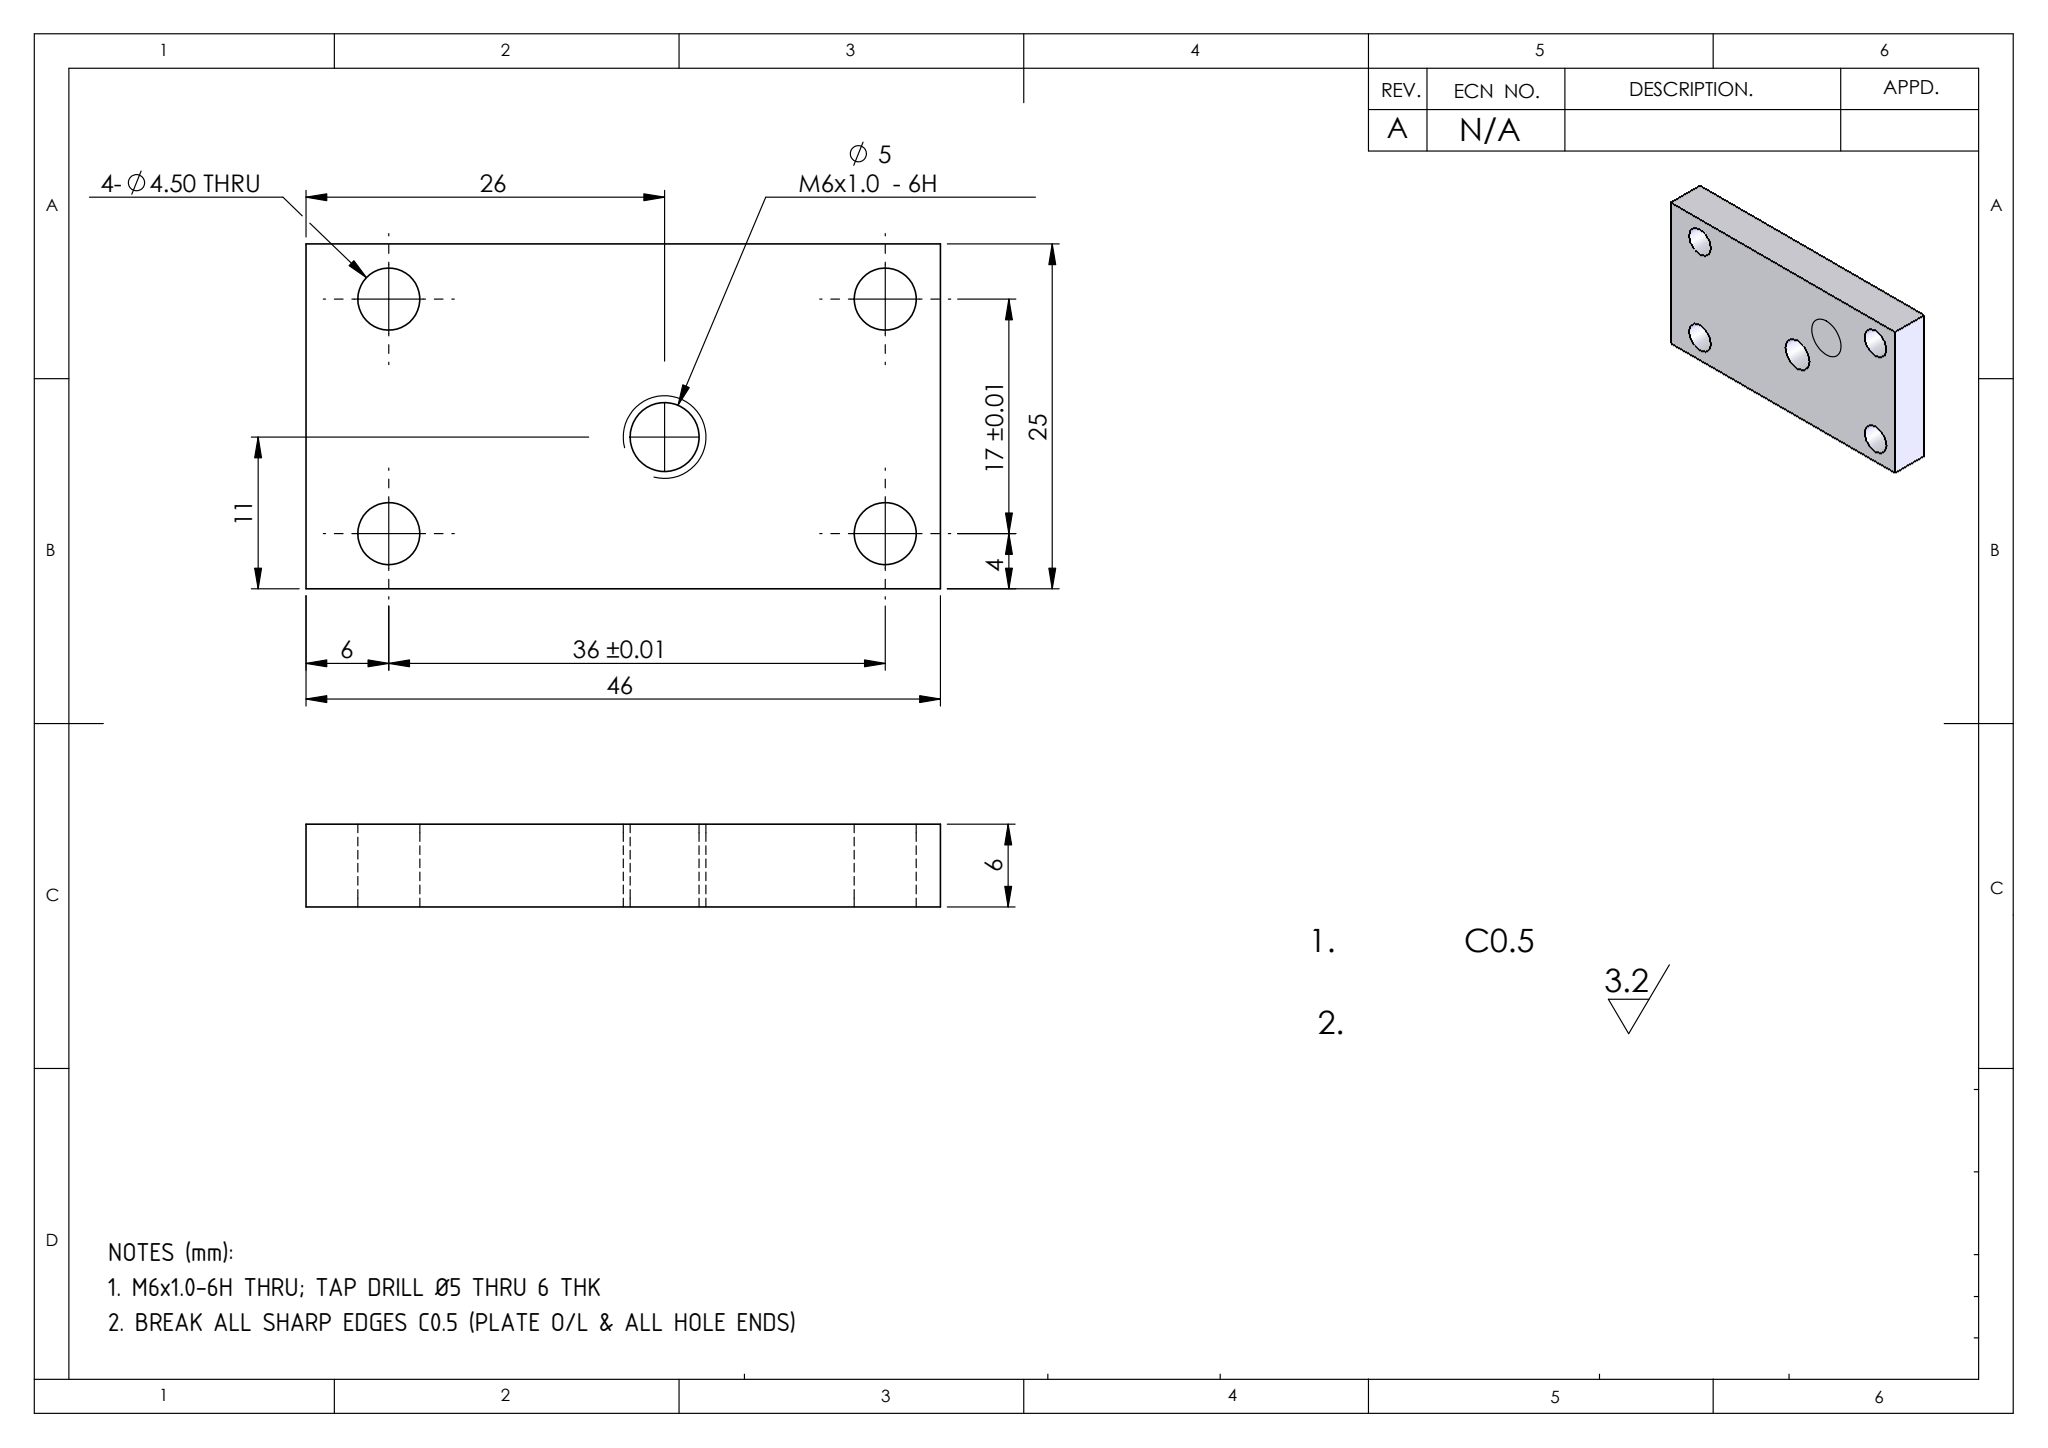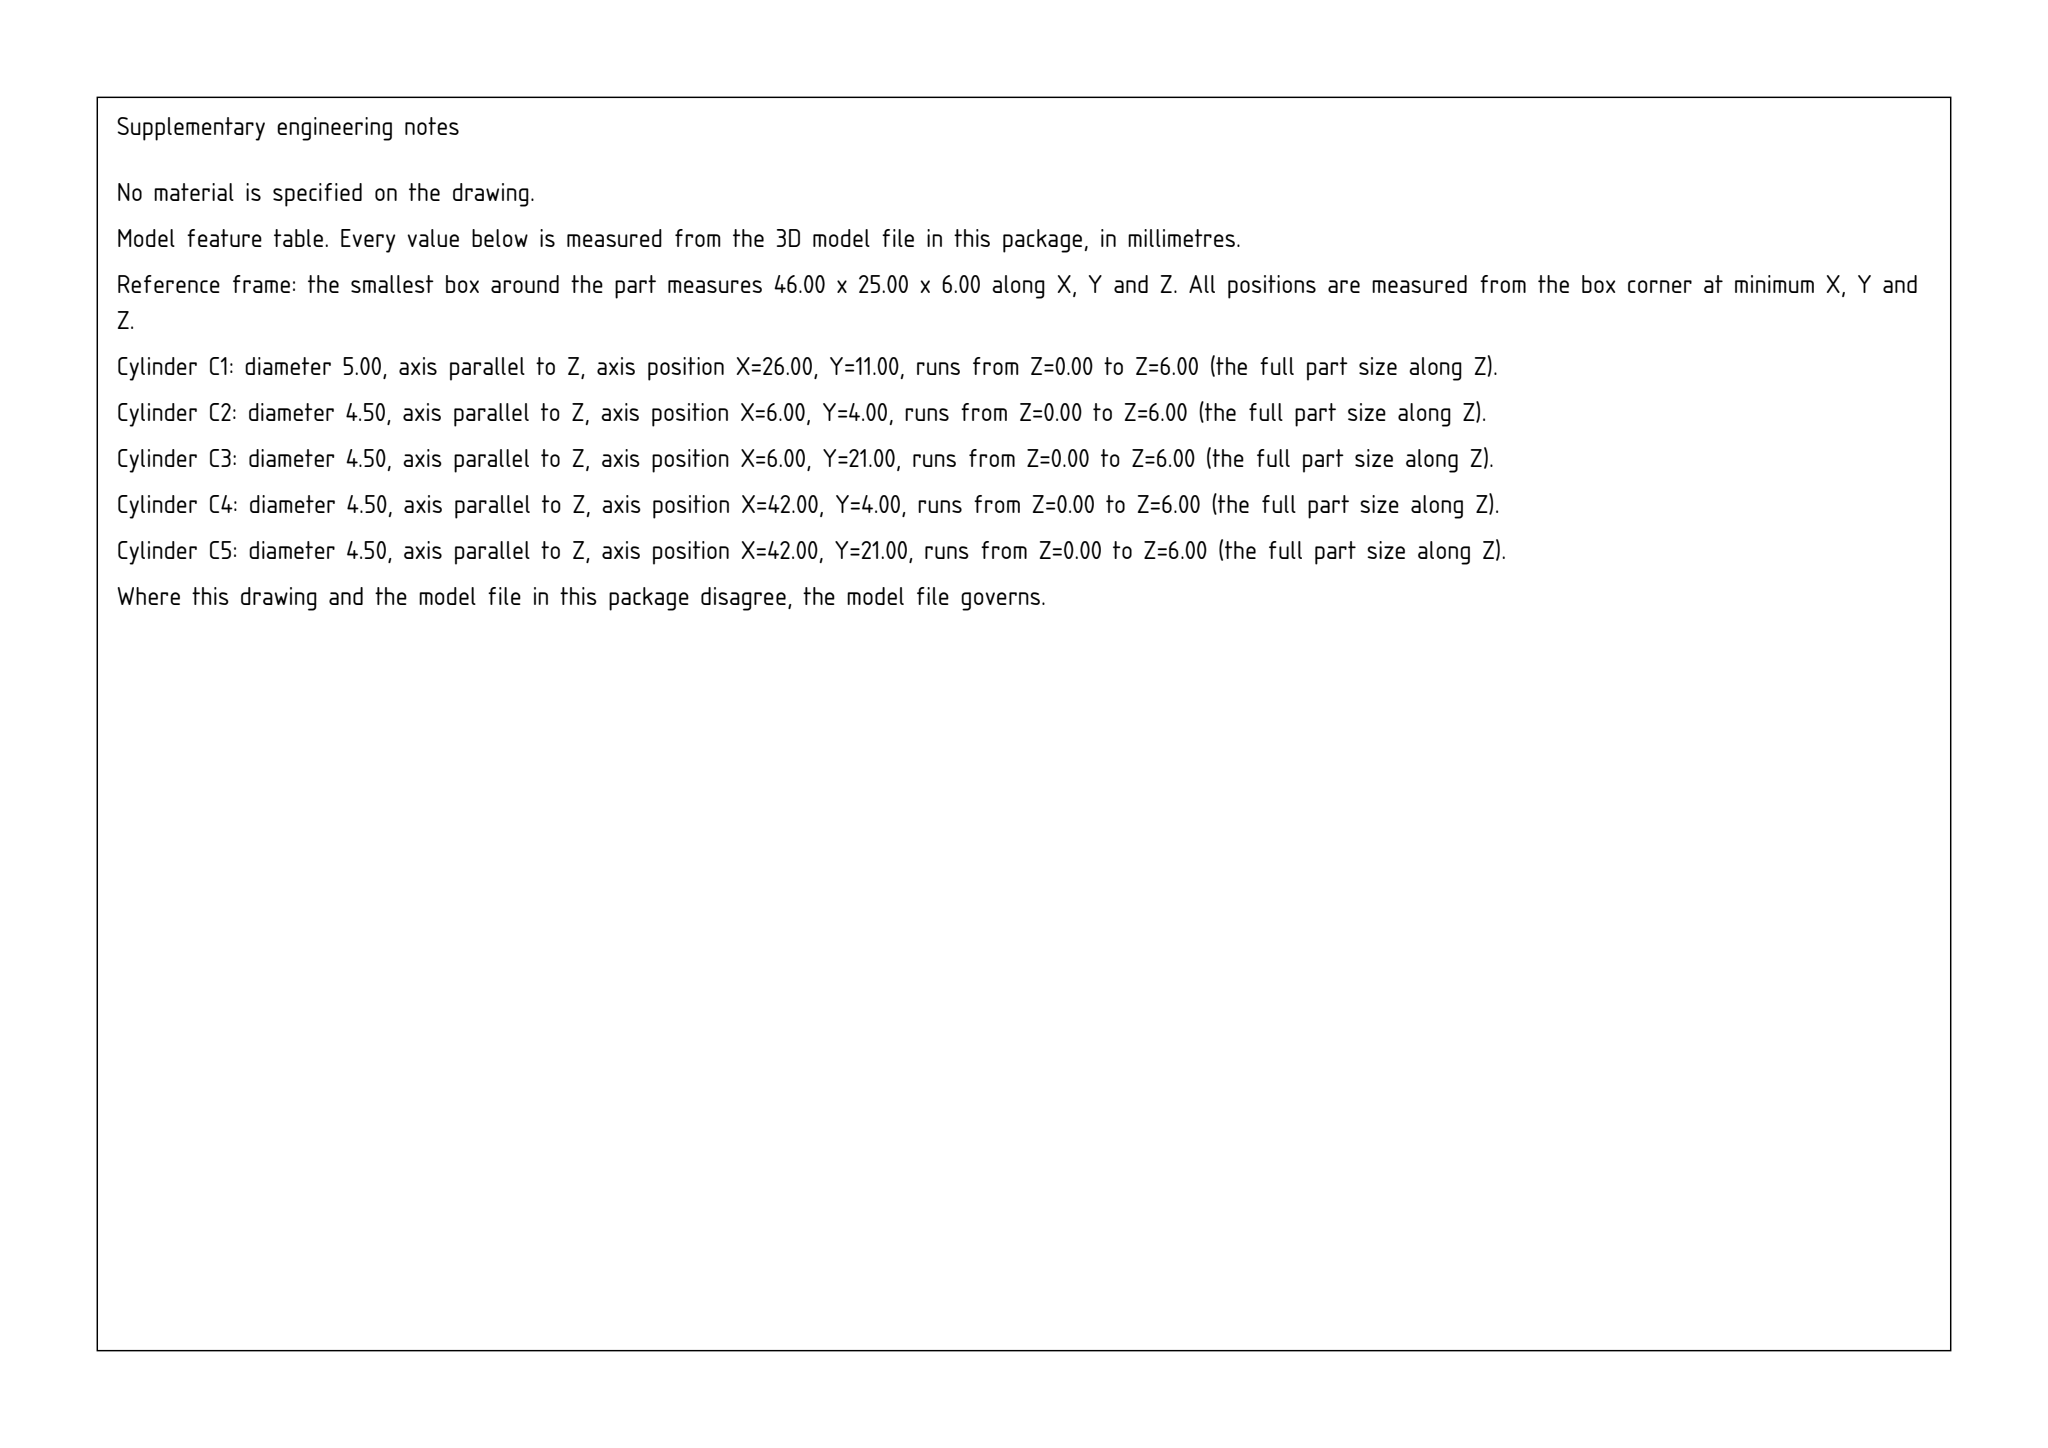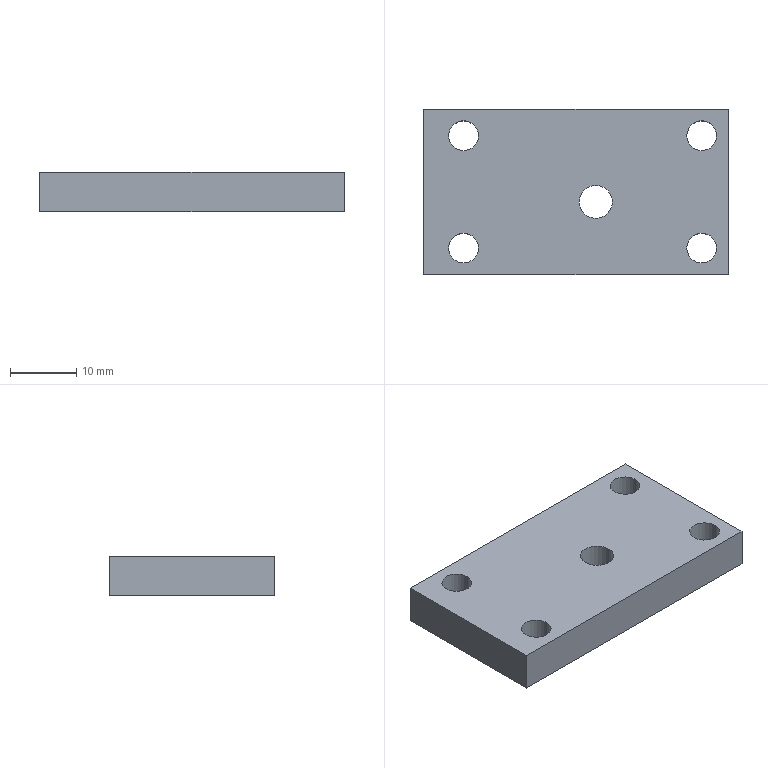Part | SolidWorks | mm | 1 solid | 16 faces | box 46 x 25 x 6 mm | volume 6400 mm3 | cylinder 10 | plane 6 | commonest cylinder face diameters 4.5 x8 5 x2
Drawing notes:
M6x1.0-6H THRU; TAP DRILL Ø5 THRU 6 THK | from the solid: Ø5 cylinder, axis z, at (26,11), length 6 = full plate thk (bbox z=6)
BREAK ALL SHARP EDGES C0.5 (PLATE O/L & ALL HOLE ENDS) | from the solid: No chamfer/fillet features in STEP; all 6 planar faces & 5 thru-hole ends meet sharp
build123d program:
from build123d import *

# Parameters (mm, degrees)
SKETCH1_W          = 46
SKETCH1_H          = 25
EXTRUDE1_DEPTH     = 6
SKETCH2_R          = 2.25
CUT_EXTRUDE1_DEPTH = 10
M6_TAPPED_HOLE1_D  = 5


with BuildPart() as part:
    # Sketch1 → Extrude1 (new body)
    with BuildSketch(Plane.XY):
        Rectangle(SKETCH1_W, SKETCH1_H)
    extrude(amount=EXTRUDE1_DEPTH)

    # Sketch2 → Cut-Extrude1 (cut)
    with BuildSketch(Plane(origin=(0, 0, 0), x_dir=(-1, 0, 0), z_dir=(0, 0, -1))):
        with Locations((-19, 8.5)):
            Circle(SKETCH2_R)
        with Locations((17, 8.5)):
            Circle(SKETCH2_R)
        with Locations((17, -8.5)):
            Circle(SKETCH2_R)
        with Locations((-19, -8.5)):
            Circle(SKETCH2_R)
    extrude(amount=-CUT_EXTRUDE1_DEPTH, mode=Mode.SUBTRACT)

    # M6 Tapped Hole1 (through all)
    with Locations(Plane(origin=(3, -1.5, 0), x_dir=(-1, 0, 0), z_dir=(0, 0, -1))):
        with Locations((0, 0)):
            Hole(M6_TAPPED_HOLE1_D / 2)


solid = part.part
STEP:
#1=CARTESIAN_POINT('',(5.5,-1.5,6.));
#2=VERTEX_POINT('',#1);
#3=CARTESIAN_POINT('',(0.5,-1.5,6.));
#4=VERTEX_POINT('',#3);
#5=CARTESIAN_POINT('',(3.,-1.5,6.));
#6=DIRECTION('',(0.,0.,-1.));
#7=DIRECTION('',(-1.,0.,0.));
#8=AXIS2_PLACEMENT_3D('',#5,#6,#7);
#9=CIRCLE('',#8,2.5);
#10=EDGE_CURVE('',#2,#4,#9,.T.);
#11=ORIENTED_EDGE('',*,*,#10,.F.);
#12=CARTESIAN_POINT('',(5.5,-1.5,0.));
#13=VERTEX_POINT('',#12);
#14=CARTESIAN_POINT('',(5.5,-1.5,-0.));
#15=DIRECTION('',(0.,0.,-1.));
#16=VECTOR('',#15,1000.);
#17=LINE('',#14,#16);
#18=EDGE_CURVE('',#2,#13,#17,.T.);
#19=ORIENTED_EDGE('',*,*,#18,.T.);
#20=CARTESIAN_POINT('',(0.5,-1.5,0.));
#21=VERTEX_POINT('',#20);
#22=CARTESIAN_POINT('',(3.,-1.5,0.));
#23=DIRECTION('',(0.,0.,-1.));
#24=DIRECTION('',(-1.,0.,0.));
#25=AXIS2_PLACEMENT_3D('',#22,#23,#24);
#26=CIRCLE('',#25,2.5);
#27=EDGE_CURVE('',#13,#21,#26,.T.);
#28=ORIENTED_EDGE('',*,*,#27,.T.);
#29=CARTESIAN_POINT('',(0.5,-1.5,0.));
#30=DIRECTION('',(0.,0.,-1.));
#31=VECTOR('',#30,1000.);
#32=LINE('',#29,#31);
#33=EDGE_CURVE('',#4,#21,#32,.T.);
#34=ORIENTED_EDGE('',*,*,#33,.F.);
#35=EDGE_LOOP('',(#11,#19,#28,#34));
#36=FACE_OUTER_BOUND('',#35,.T.);
#37=CARTESIAN_POINT('',(3.,-1.5,0.));
#38=DIRECTION('',(0.,0.,-1.));
#39=DIRECTION('',(-1.,0.,0.));
#40=AXIS2_PLACEMENT_3D('',#37,#38,#39);
#41=CYLINDRICAL_SURFACE('',#40,2.5);
#42=ADVANCED_FACE('',(#36),#41,.F.);
#43=CARTESIAN_POINT('',(21.25,-8.5,6.));
#44=VERTEX_POINT('',#43);
#45=CARTESIAN_POINT('',(16.75,-8.5,6.));
#46=VERTEX_POINT('',#45);
#47=CARTESIAN_POINT('',(19.,-8.5,6.));
#48=DIRECTION('',(0.,0.,-1.));
#49=DIRECTION('',(-1.,0.,0.));
#50=AXIS2_PLACEMENT_3D('',#47,#48,#49);
#51=CIRCLE('',#50,2.25);
#52=EDGE_CURVE('',#44,#46,#51,.T.);
#53=ORIENTED_EDGE('',*,*,#52,.F.);
#54=CARTESIAN_POINT('',(21.25,-8.5,0.));
#55=VERTEX_POINT('',#54);
#56=CARTESIAN_POINT('',(21.25,-8.5,10.));
#57=DIRECTION('',(0.,0.,-1.));
#58=VECTOR('',#57,1000.);
#59=LINE('',#56,#58);
#60=EDGE_CURVE('',#44,#55,#59,.T.);
#61=ORIENTED_EDGE('',*,*,#60,.T.);
#62=CARTESIAN_POINT('',(16.75,-8.5,-0.));
#63=VERTEX_POINT('',#62);
#64=CARTESIAN_POINT('',(19.,-8.5,0.));
#65=DIRECTION('',(0.,0.,-1.));
#66=DIRECTION('',(1.,0.,-0.));
#67=AXIS2_PLACEMENT_3D('',#64,#65,#66);
#68=CIRCLE('',#67,2.25);
#69=EDGE_CURVE('',#55,#63,#68,.T.);
#70=ORIENTED_EDGE('',*,*,#69,.T.);
#71=CARTESIAN_POINT('',(16.75,-8.5,10.));
#72=DIRECTION('',(0.,0.,-1.));
#73=VECTOR('',#72,1000.);
#74=LINE('',#71,#73);
#75=EDGE_CURVE('',#46,#63,#74,.T.);
#76=ORIENTED_EDGE('',*,*,#75,.F.);
#77=EDGE_LOOP('',(#53,#61,#70,#76));
#78=FACE_OUTER_BOUND('',#77,.T.);
#79=CARTESIAN_POINT('',(19.,-8.5,10.));
#80=DIRECTION('',(0.,0.,-1.));
#81=DIRECTION('',(-1.,0.,0.));
#82=AXIS2_PLACEMENT_3D('',#79,#80,#81);
#83=CYLINDRICAL_SURFACE('',#82,2.25);
#84=ADVANCED_FACE('',(#78),#83,.F.);
#85=CARTESIAN_POINT('',(-14.75,-8.5,6.));
#86=VERTEX_POINT('',#85);
#87=CARTESIAN_POINT('',(-19.25,-8.5,6.));
#88=VERTEX_POINT('',#87);
#89=CARTESIAN_POINT('',(-17.,-8.5,6.));
#90=DIRECTION('',(0.,0.,-1.));
#91=DIRECTION('',(-1.,0.,0.));
#92=AXIS2_PLACEMENT_3D('',#89,#90,#91);
#93=CIRCLE('',#92,2.25);
#94=EDGE_CURVE('',#86,#88,#93,.T.);
#95=ORIENTED_EDGE('',*,*,#94,.F.);
#96=CARTESIAN_POINT('',(-14.75,-8.5,0.));
#97=VERTEX_POINT('',#96);
#98=CARTESIAN_POINT('',(-14.75,-8.5,10.));
#99=DIRECTION('',(0.,0.,-1.));
#100=VECTOR('',#99,1000.);
#101=LINE('',#98,#100);
#102=EDGE_CURVE('',#86,#97,#101,.T.);
#103=ORIENTED_EDGE('',*,*,#102,.T.);
#104=CARTESIAN_POINT('',(-19.25,-8.5,0.));
#105=VERTEX_POINT('',#104);
#106=CARTESIAN_POINT('',(-17.,-8.5,0.));
#107=DIRECTION('',(0.,0.,-1.));
#108=DIRECTION('',(1.,0.,-0.));
#109=AXIS2_PLACEMENT_3D('',#106,#107,#108);
#110=CIRCLE('',#109,2.25);
#111=EDGE_CURVE('',#97,#105,#110,.T.);
#112=ORIENTED_EDGE('',*,*,#111,.T.);
#113=CARTESIAN_POINT('',(-19.25,-8.5,10.));
#114=DIRECTION('',(0.,0.,-1.));
#115=VECTOR('',#114,1000.);
#116=LINE('',#113,#115);
#117=EDGE_CURVE('',#88,#105,#116,.T.);
#118=ORIENTED_EDGE('',*,*,#117,.F.);
#119=EDGE_LOOP('',(#95,#103,#112,#118));
#120=FACE_OUTER_BOUND('',#119,.T.);
#121=CARTESIAN_POINT('',(-17.,-8.5,10.));
#122=DIRECTION('',(0.,0.,-1.));
#123=DIRECTION('',(-1.,0.,0.));
#124=AXIS2_PLACEMENT_3D('',#121,#122,#123);
#125=CYLINDRICAL_SURFACE('',#124,2.25);
#126=ADVANCED_FACE('',(#120),#125,.F.);
#127=CARTESIAN_POINT('',(-14.75,8.5,6.));
#128=VERTEX_POINT('',#127);
#129=CARTESIAN_POINT('',(-19.25,8.5,6.));
#130=VERTEX_POINT('',#129);
#131=CARTESIAN_POINT('',(-17.,8.5,6.));
#132=DIRECTION('',(0.,0.,-1.));
#133=DIRECTION('',(-1.,0.,0.));
#134=AXIS2_PLACEMENT_3D('',#131,#132,#133);
#135=CIRCLE('',#134,2.25);
#136=EDGE_CURVE('',#128,#130,#135,.T.);
#137=ORIENTED_EDGE('',*,*,#136,.F.);
#138=CARTESIAN_POINT('',(-14.75,8.5,0.));
#139=VERTEX_POINT('',#138);
#140=CARTESIAN_POINT('',(-14.75,8.5,10.));
#141=DIRECTION('',(0.,0.,-1.));
#142=VECTOR('',#141,1000.);
#143=LINE('',#140,#142);
#144=EDGE_CURVE('',#128,#139,#143,.T.);
#145=ORIENTED_EDGE('',*,*,#144,.T.);
#146=CARTESIAN_POINT('',(-19.25,8.5,0.));
#147=VERTEX_POINT('',#146);
#148=CARTESIAN_POINT('',(-17.,8.5,0.));
#149=DIRECTION('',(0.,0.,-1.));
#150=DIRECTION('',(-1.,0.,0.));
#151=AXIS2_PLACEMENT_3D('',#148,#149,#150);
#152=CIRCLE('',#151,2.25);
#153=EDGE_CURVE('',#139,#147,#152,.T.);
#154=ORIENTED_EDGE('',*,*,#153,.T.);
#155=CARTESIAN_POINT('',(-19.25,8.5,10.));
#156=DIRECTION('',(0.,0.,-1.));
#157=VECTOR('',#156,1000.);
#158=LINE('',#155,#157);
#159=EDGE_CURVE('',#130,#147,#158,.T.);
#160=ORIENTED_EDGE('',*,*,#159,.F.);
#161=EDGE_LOOP('',(#137,#145,#154,#160));
#162=FACE_OUTER_BOUND('',#161,.T.);
#163=CARTESIAN_POINT('',(-17.,8.5,10.));
#164=DIRECTION('',(0.,0.,-1.));
#165=DIRECTION('',(-1.,0.,0.));
#166=AXIS2_PLACEMENT_3D('',#163,#164,#165);
#167=CYLINDRICAL_SURFACE('',#166,2.25);
#168=ADVANCED_FACE('',(#162),#167,.F.);
#169=CARTESIAN_POINT('',(21.25,8.5,6.));
#170=VERTEX_POINT('',#169);
#171=CARTESIAN_POINT('',(16.75,8.5,6.));
#172=VERTEX_POINT('',#171);
#173=CARTESIAN_POINT('',(19.,8.5,6.));
#174=DIRECTION('',(0.,0.,-1.));
#175=DIRECTION('',(-1.,0.,0.));
#176=AXIS2_PLACEMENT_3D('',#173,#174,#175);
#177=CIRCLE('',#176,2.25);
#178=EDGE_CURVE('',#170,#172,#177,.T.);
#179=ORIENTED_EDGE('',*,*,#178,.F.);
#180=CARTESIAN_POINT('',(21.25,8.5,0.));
#181=VERTEX_POINT('',#180);
#182=CARTESIAN_POINT('',(21.25,8.5,10.));
#183=DIRECTION('',(0.,0.,-1.));
#184=VECTOR('',#183,1000.);
#185=LINE('',#182,#184);
#186=EDGE_CURVE('',#170,#181,#185,.T.);
#187=ORIENTED_EDGE('',*,*,#186,.T.);
#188=CARTESIAN_POINT('',(16.75,8.5,0.));
#189=VERTEX_POINT('',#188);
#190=CARTESIAN_POINT('',(19.,8.5,0.));
#191=DIRECTION('',(0.,0.,-1.));
#192=DIRECTION('',(-1.,0.,0.));
#193=AXIS2_PLACEMENT_3D('',#190,#191,#192);
#194=CIRCLE('',#193,2.25);
#195=EDGE_CURVE('',#181,#189,#194,.T.);
#196=ORIENTED_EDGE('',*,*,#195,.T.);
#197=CARTESIAN_POINT('',(16.75,8.5,10.));
#198=DIRECTION('',(0.,0.,-1.));
#199=VECTOR('',#198,1000.);
#200=LINE('',#197,#199);
#201=EDGE_CURVE('',#172,#189,#200,.T.);
#202=ORIENTED_EDGE('',*,*,#201,.F.);
#203=EDGE_LOOP('',(#179,#187,#196,#202));
#204=FACE_OUTER_BOUND('',#203,.T.);
#205=CARTESIAN_POINT('',(19.,8.5,10.));
#206=DIRECTION('',(0.,0.,-1.));
#207=DIRECTION('',(-1.,0.,0.));
#208=AXIS2_PLACEMENT_3D('',#205,#206,#207);
#209=CYLINDRICAL_SURFACE('',#208,2.25);
#210=ADVANCED_FACE('',(#204),#209,.F.);
#211=CARTESIAN_POINT('',(23.,-12.5,0.));
#212=VERTEX_POINT('',#211);
#213=CARTESIAN_POINT('',(23.,12.5,0.));
#214=VERTEX_POINT('',#213);
#215=CARTESIAN_POINT('',(23.,12.5,0.));
#216=DIRECTION('',(0.,1.,0.));
#217=VECTOR('',#216,1000.);
#218=LINE('',#215,#217);
#219=EDGE_CURVE('',#212,#214,#218,.T.);
#220=ORIENTED_EDGE('',*,*,#219,.T.);
#221=CARTESIAN_POINT('',(23.,12.5,6.));
#222=VERTEX_POINT('',#221);
#223=CARTESIAN_POINT('',(23.,12.5,6.));
#224=DIRECTION('',(0.,0.,-1.));
#225=VECTOR('',#224,1000.);
#226=LINE('',#223,#225);
#227=EDGE_CURVE('',#222,#214,#226,.T.);
#228=ORIENTED_EDGE('',*,*,#227,.F.);
#229=CARTESIAN_POINT('',(23.,-12.5,6.));
#230=VERTEX_POINT('',#229);
#231=CARTESIAN_POINT('',(23.,12.5,6.));
#232=DIRECTION('',(0.,1.,0.));
#233=VECTOR('',#232,1000.);
#234=LINE('',#231,#233);
#235=EDGE_CURVE('',#230,#222,#234,.T.);
#236=ORIENTED_EDGE('',*,*,#235,.F.);
#237=CARTESIAN_POINT('',(23.,-12.5,6.));
#238=DIRECTION('',(0.,0.,-1.));
#239=VECTOR('',#238,1000.);
#240=LINE('',#237,#239);
#241=EDGE_CURVE('',#230,#212,#240,.T.);
#242=ORIENTED_EDGE('',*,*,#241,.T.);
#243=EDGE_LOOP('',(#220,#228,#236,#242));
#244=FACE_OUTER_BOUND('',#243,.T.);
#245=CARTESIAN_POINT('',(23.,12.5,6.));
#246=DIRECTION('',(-1.,0.,0.));
#247=DIRECTION('',(-0.,-1.,0.));
#248=AXIS2_PLACEMENT_3D('',#245,#246,#247);
#249=PLANE('',#248);
#250=ADVANCED_FACE('',(#244),#249,.F.);
#251=CARTESIAN_POINT('',(-23.,12.5,0.));
#252=VERTEX_POINT('',#251);
#253=CARTESIAN_POINT('',(23.,12.5,0.));
#254=DIRECTION('',(-1.,0.,0.));
#255=VECTOR('',#254,1000.);
#256=LINE('',#253,#255);
#257=EDGE_CURVE('',#214,#252,#256,.T.);
#258=ORIENTED_EDGE('',*,*,#257,.T.);
#259=CARTESIAN_POINT('',(-23.,12.5,6.));
#260=VERTEX_POINT('',#259);
#261=CARTESIAN_POINT('',(-23.,12.5,6.));
#262=DIRECTION('',(0.,0.,-1.));
#263=VECTOR('',#262,1000.);
#264=LINE('',#261,#263);
#265=EDGE_CURVE('',#260,#252,#264,.T.);
#266=ORIENTED_EDGE('',*,*,#265,.F.);
#267=CARTESIAN_POINT('',(23.,12.5,6.));
#268=DIRECTION('',(-1.,0.,0.));
#269=VECTOR('',#268,1000.);
#270=LINE('',#267,#269);
#271=EDGE_CURVE('',#222,#260,#270,.T.);
#272=ORIENTED_EDGE('',*,*,#271,.F.);
#273=ORIENTED_EDGE('',*,*,#227,.T.);
#274=EDGE_LOOP('',(#258,#266,#272,#273));
#275=FACE_OUTER_BOUND('',#274,.T.);
#276=CARTESIAN_POINT('',(23.,12.5,6.));
#277=DIRECTION('',(-0.,-1.,-0.));
#278=DIRECTION('',(1.,-0.,-0.));
#279=AXIS2_PLACEMENT_3D('',#276,#277,#278);
#280=PLANE('',#279);
#281=ADVANCED_FACE('',(#275),#280,.F.);
#282=CARTESIAN_POINT('',(-23.,-12.5,0.));
#283=VERTEX_POINT('',#282);
#284=CARTESIAN_POINT('',(-23.,12.5,0.));
#285=DIRECTION('',(-0.,-1.,0.));
#286=VECTOR('',#285,1000.);
#287=LINE('',#284,#286);
#288=EDGE_CURVE('',#252,#283,#287,.T.);
#289=ORIENTED_EDGE('',*,*,#288,.T.);
#290=CARTESIAN_POINT('',(-23.,-12.5,6.));
#291=VERTEX_POINT('',#290);
#292=CARTESIAN_POINT('',(-23.,-12.5,6.));
#293=DIRECTION('',(0.,0.,-1.));
#294=VECTOR('',#293,1000.);
#295=LINE('',#292,#294);
#296=EDGE_CURVE('',#291,#283,#295,.T.);
#297=ORIENTED_EDGE('',*,*,#296,.F.);
#298=CARTESIAN_POINT('',(-23.,12.5,6.));
#299=DIRECTION('',(-0.,-1.,0.));
#300=VECTOR('',#299,1000.);
#301=LINE('',#298,#300);
#302=EDGE_CURVE('',#260,#291,#301,.T.);
#303=ORIENTED_EDGE('',*,*,#302,.F.);
#304=ORIENTED_EDGE('',*,*,#265,.T.);
#305=EDGE_LOOP('',(#289,#297,#303,#304));
#306=FACE_OUTER_BOUND('',#305,.T.);
#307=CARTESIAN_POINT('',(-23.,12.5,6.));
#308=DIRECTION('',(1.,-0.,-0.));
#309=DIRECTION('',(0.,1.,0.));
#310=AXIS2_PLACEMENT_3D('',#307,#308,#309);
#311=PLANE('',#310);
#312=ADVANCED_FACE('',(#306),#311,.F.);
#313=CARTESIAN_POINT('',(23.,-12.5,0.));
#314=DIRECTION('',(1.,0.,-0.));
#315=VECTOR('',#314,1000.);
#316=LINE('',#313,#315);
#317=EDGE_CURVE('',#283,#212,#316,.T.);
#318=ORIENTED_EDGE('',*,*,#317,.T.);
#319=ORIENTED_EDGE('',*,*,#241,.F.);
#320=CARTESIAN_POINT('',(23.,-12.5,6.));
#321=DIRECTION('',(1.,0.,-0.));
#322=VECTOR('',#321,1000.);
#323=LINE('',#320,#322);
#324=EDGE_CURVE('',#291,#230,#323,.T.);
#325=ORIENTED_EDGE('',*,*,#324,.F.);
#326=ORIENTED_EDGE('',*,*,#296,.T.);
#327=EDGE_LOOP('',(#318,#319,#325,#326));
#328=FACE_OUTER_BOUND('',#327,.T.);
#329=CARTESIAN_POINT('',(23.,-12.5,6.));
#330=DIRECTION('',(-0.,1.,0.));
#331=DIRECTION('',(-1.,-0.,0.));
#332=AXIS2_PLACEMENT_3D('',#329,#330,#331);
#333=PLANE('',#332);
#334=ADVANCED_FACE('',(#328),#333,.F.);
#335=CARTESIAN_POINT('',(3.,-1.5,6.));
#336=DIRECTION('',(0.,0.,-1.));
#337=DIRECTION('',(-1.,0.,0.));
#338=AXIS2_PLACEMENT_3D('',#335,#336,#337);
#339=CIRCLE('',#338,2.5);
#340=EDGE_CURVE('',#4,#2,#339,.T.);
#341=ORIENTED_EDGE('',*,*,#340,.T.);
#342=ORIENTED_EDGE('',*,*,#10,.T.);
#343=EDGE_LOOP('',(#341,#342));
#344=FACE_BOUND('',#343,.T.);
#345=CARTESIAN_POINT('',(19.,-8.5,6.));
#346=DIRECTION('',(0.,0.,-1.));
#347=DIRECTION('',(-1.,0.,0.));
#348=AXIS2_PLACEMENT_3D('',#345,#346,#347);
#349=CIRCLE('',#348,2.25);
#350=EDGE_CURVE('',#46,#44,#349,.T.);
#351=ORIENTED_EDGE('',*,*,#350,.T.);
#352=ORIENTED_EDGE('',*,*,#52,.T.);
#353=EDGE_LOOP('',(#351,#352));
#354=FACE_BOUND('',#353,.T.);
#355=CARTESIAN_POINT('',(-17.,-8.5,6.));
#356=DIRECTION('',(0.,0.,-1.));
#357=DIRECTION('',(-1.,0.,0.));
#358=AXIS2_PLACEMENT_3D('',#355,#356,#357);
#359=CIRCLE('',#358,2.25);
#360=EDGE_CURVE('',#88,#86,#359,.T.);
#361=ORIENTED_EDGE('',*,*,#360,.T.);
#362=ORIENTED_EDGE('',*,*,#94,.T.);
#363=EDGE_LOOP('',(#361,#362));
#364=FACE_BOUND('',#363,.T.);
#365=CARTESIAN_POINT('',(-17.,8.5,6.));
#366=DIRECTION('',(0.,0.,-1.));
#367=DIRECTION('',(-1.,0.,0.));
#368=AXIS2_PLACEMENT_3D('',#365,#366,#367);
#369=CIRCLE('',#368,2.25);
#370=EDGE_CURVE('',#130,#128,#369,.T.);
#371=ORIENTED_EDGE('',*,*,#370,.T.);
#372=ORIENTED_EDGE('',*,*,#136,.T.);
#373=EDGE_LOOP('',(#371,#372));
#374=FACE_BOUND('',#373,.T.);
#375=CARTESIAN_POINT('',(19.,8.5,6.));
#376=DIRECTION('',(0.,0.,-1.));
#377=DIRECTION('',(-1.,0.,0.));
#378=AXIS2_PLACEMENT_3D('',#375,#376,#377);
#379=CIRCLE('',#378,2.25);
#380=EDGE_CURVE('',#172,#170,#379,.T.);
#381=ORIENTED_EDGE('',*,*,#380,.T.);
#382=ORIENTED_EDGE('',*,*,#178,.T.);
#383=EDGE_LOOP('',(#381,#382));
#384=FACE_BOUND('',#383,.T.);
#385=ORIENTED_EDGE('',*,*,#235,.T.);
#386=ORIENTED_EDGE('',*,*,#271,.T.);
#387=ORIENTED_EDGE('',*,*,#302,.T.);
#388=ORIENTED_EDGE('',*,*,#324,.T.);
#389=EDGE_LOOP('',(#385,#386,#387,#388));
#390=FACE_OUTER_BOUND('',#389,.T.);
#391=CARTESIAN_POINT('',(23.,12.5,6.));
#392=DIRECTION('',(-0.,-0.,-1.));
#393=DIRECTION('',(-1.,-0.,0.));
#394=AXIS2_PLACEMENT_3D('',#391,#392,#393);
#395=PLANE('',#394);
#396=ADVANCED_FACE('',(#344,#354,#364,#374,#384,#390),#395,.F.);
#397=CARTESIAN_POINT('',(3.,-1.5,0.));
#398=DIRECTION('',(0.,0.,-1.));
#399=DIRECTION('',(-1.,0.,0.));
#400=AXIS2_PLACEMENT_3D('',#397,#398,#399);
#401=CIRCLE('',#400,2.5);
#402=EDGE_CURVE('',#21,#13,#401,.T.);
#403=ORIENTED_EDGE('',*,*,#402,.F.);
#404=ORIENTED_EDGE('',*,*,#27,.F.);
#405=EDGE_LOOP('',(#403,#404));
#406=FACE_BOUND('',#405,.T.);
#407=CARTESIAN_POINT('',(19.,-8.5,0.));
#408=DIRECTION('',(0.,0.,-1.));
#409=DIRECTION('',(1.,0.,-0.));
#410=AXIS2_PLACEMENT_3D('',#407,#408,#409);
#411=CIRCLE('',#410,2.25);
#412=EDGE_CURVE('',#63,#55,#411,.T.);
#413=ORIENTED_EDGE('',*,*,#412,.F.);
#414=ORIENTED_EDGE('',*,*,#69,.F.);
#415=EDGE_LOOP('',(#413,#414));
#416=FACE_BOUND('',#415,.T.);
#417=CARTESIAN_POINT('',(-17.,-8.5,0.));
#418=DIRECTION('',(0.,0.,-1.));
#419=DIRECTION('',(1.,0.,-0.));
#420=AXIS2_PLACEMENT_3D('',#417,#418,#419);
#421=CIRCLE('',#420,2.25);
#422=EDGE_CURVE('',#105,#97,#421,.T.);
#423=ORIENTED_EDGE('',*,*,#422,.F.);
#424=ORIENTED_EDGE('',*,*,#111,.F.);
#425=EDGE_LOOP('',(#423,#424));
#426=FACE_BOUND('',#425,.T.);
#427=CARTESIAN_POINT('',(-17.,8.5,0.));
#428=DIRECTION('',(0.,0.,-1.));
#429=DIRECTION('',(-1.,0.,0.));
#430=AXIS2_PLACEMENT_3D('',#427,#428,#429);
#431=CIRCLE('',#430,2.25);
#432=EDGE_CURVE('',#147,#139,#431,.T.);
#433=ORIENTED_EDGE('',*,*,#432,.F.);
#434=ORIENTED_EDGE('',*,*,#153,.F.);
#435=EDGE_LOOP('',(#433,#434));
#436=FACE_BOUND('',#435,.T.);
#437=CARTESIAN_POINT('',(19.,8.5,0.));
#438=DIRECTION('',(0.,0.,-1.));
#439=DIRECTION('',(-1.,0.,0.));
#440=AXIS2_PLACEMENT_3D('',#437,#438,#439);
#441=CIRCLE('',#440,2.25);
#442=EDGE_CURVE('',#189,#181,#441,.T.);
#443=ORIENTED_EDGE('',*,*,#442,.F.);
#444=ORIENTED_EDGE('',*,*,#195,.F.);
#445=EDGE_LOOP('',(#443,#444));
#446=FACE_BOUND('',#445,.T.);
#447=ORIENTED_EDGE('',*,*,#219,.F.);
#448=ORIENTED_EDGE('',*,*,#317,.F.);
#449=ORIENTED_EDGE('',*,*,#288,.F.);
#450=ORIENTED_EDGE('',*,*,#257,.F.);
#451=EDGE_LOOP('',(#447,#448,#449,#450));
#452=FACE_OUTER_BOUND('',#451,.T.);
#453=CARTESIAN_POINT('',(23.,12.5,0.));
#454=DIRECTION('',(-0.,-0.,-1.));
#455=DIRECTION('',(-1.,-0.,0.));
#456=AXIS2_PLACEMENT_3D('',#453,#454,#455);
#457=PLANE('',#456);
#458=ADVANCED_FACE('',(#406,#416,#426,#436,#446,#452),#457,.T.);
#459=ORIENTED_EDGE('',*,*,#186,.F.);
#460=ORIENTED_EDGE('',*,*,#380,.F.);
#461=ORIENTED_EDGE('',*,*,#201,.T.);
#462=ORIENTED_EDGE('',*,*,#442,.T.);
#463=EDGE_LOOP('',(#459,#460,#461,#462));
#464=FACE_OUTER_BOUND('',#463,.T.);
#465=CARTESIAN_POINT('',(19.,8.5,10.));
#466=DIRECTION('',(0.,0.,-1.));
#467=DIRECTION('',(-1.,0.,0.));
#468=AXIS2_PLACEMENT_3D('',#465,#466,#467);
#469=CYLINDRICAL_SURFACE('',#468,2.25);
#470=ADVANCED_FACE('',(#464),#469,.F.);
#471=ORIENTED_EDGE('',*,*,#144,.F.);
#472=ORIENTED_EDGE('',*,*,#370,.F.);
#473=ORIENTED_EDGE('',*,*,#159,.T.);
#474=ORIENTED_EDGE('',*,*,#432,.T.);
#475=EDGE_LOOP('',(#471,#472,#473,#474));
#476=FACE_OUTER_BOUND('',#475,.T.);
#477=CARTESIAN_POINT('',(-17.,8.5,10.));
#478=DIRECTION('',(0.,0.,-1.));
#479=DIRECTION('',(-1.,0.,0.));
#480=AXIS2_PLACEMENT_3D('',#477,#478,#479);
#481=CYLINDRICAL_SURFACE('',#480,2.25);
#482=ADVANCED_FACE('',(#476),#481,.F.);
#483=ORIENTED_EDGE('',*,*,#102,.F.);
#484=ORIENTED_EDGE('',*,*,#360,.F.);
#485=ORIENTED_EDGE('',*,*,#117,.T.);
#486=ORIENTED_EDGE('',*,*,#422,.T.);
#487=EDGE_LOOP('',(#483,#484,#485,#486));
#488=FACE_OUTER_BOUND('',#487,.T.);
#489=CARTESIAN_POINT('',(-17.,-8.5,10.));
#490=DIRECTION('',(0.,0.,-1.));
#491=DIRECTION('',(-1.,0.,0.));
#492=AXIS2_PLACEMENT_3D('',#489,#490,#491);
#493=CYLINDRICAL_SURFACE('',#492,2.25);
#494=ADVANCED_FACE('',(#488),#493,.F.);
#495=ORIENTED_EDGE('',*,*,#60,.F.);
#496=ORIENTED_EDGE('',*,*,#350,.F.);
#497=ORIENTED_EDGE('',*,*,#75,.T.);
#498=ORIENTED_EDGE('',*,*,#412,.T.);
#499=EDGE_LOOP('',(#495,#496,#497,#498));
#500=FACE_OUTER_BOUND('',#499,.T.);
#501=CARTESIAN_POINT('',(19.,-8.5,10.));
#502=DIRECTION('',(0.,0.,-1.));
#503=DIRECTION('',(-1.,0.,0.));
#504=AXIS2_PLACEMENT_3D('',#501,#502,#503);
#505=CYLINDRICAL_SURFACE('',#504,2.25);
#506=ADVANCED_FACE('',(#500),#505,.F.);
#507=ORIENTED_EDGE('',*,*,#18,.F.);
#508=ORIENTED_EDGE('',*,*,#340,.F.);
#509=ORIENTED_EDGE('',*,*,#33,.T.);
#510=ORIENTED_EDGE('',*,*,#402,.T.);
#511=EDGE_LOOP('',(#507,#508,#509,#510));
#512=FACE_OUTER_BOUND('',#511,.T.);
#513=CARTESIAN_POINT('',(3.,-1.5,0.));
#514=DIRECTION('',(0.,0.,-1.));
#515=DIRECTION('',(-1.,0.,0.));
#516=AXIS2_PLACEMENT_3D('',#513,#514,#515);
#517=CYLINDRICAL_SURFACE('',#516,2.5);
#518=ADVANCED_FACE('',(#512),#517,.F.);
#519=CLOSED_SHELL('',(#42,#84,#126,#168,#210,#250,#281,#312,#334,#396,#458,#470,#482,#494,#506,#518));
#520=MANIFOLD_SOLID_BREP('',#519);
#521=CARTESIAN_POINT('',(0.,0.,0.));
#522=DIRECTION('',(0.,0.,1.));
#523=DIRECTION('',(1.,0.,0.));
#524=AXIS2_PLACEMENT_3D('',#521,#522,#523);
#525=(LENGTH_UNIT()NAMED_UNIT(*)SI_UNIT(.MILLI.,.METRE.));
#526=UNCERTAINTY_MEASURE_WITH_UNIT(LENGTH_MEASURE(0.00001),#525,'','');
#527=(NAMED_UNIT(*)PLANE_ANGLE_UNIT()SI_UNIT($,.RADIAN.));
#528=(NAMED_UNIT(*)SI_UNIT($,.STERADIAN.)SOLID_ANGLE_UNIT());
#529=(GEOMETRIC_REPRESENTATION_CONTEXT(3)GLOBAL_UNCERTAINTY_ASSIGNED_CONTEXT((#526))GLOBAL_UNIT_ASSIGNED_CONTEXT((#525,#527,#528))REPRESENTATION_CONTEXT('',''));
#530=ADVANCED_BREP_SHAPE_REPRESENTATION('',(#520,#524),#529);